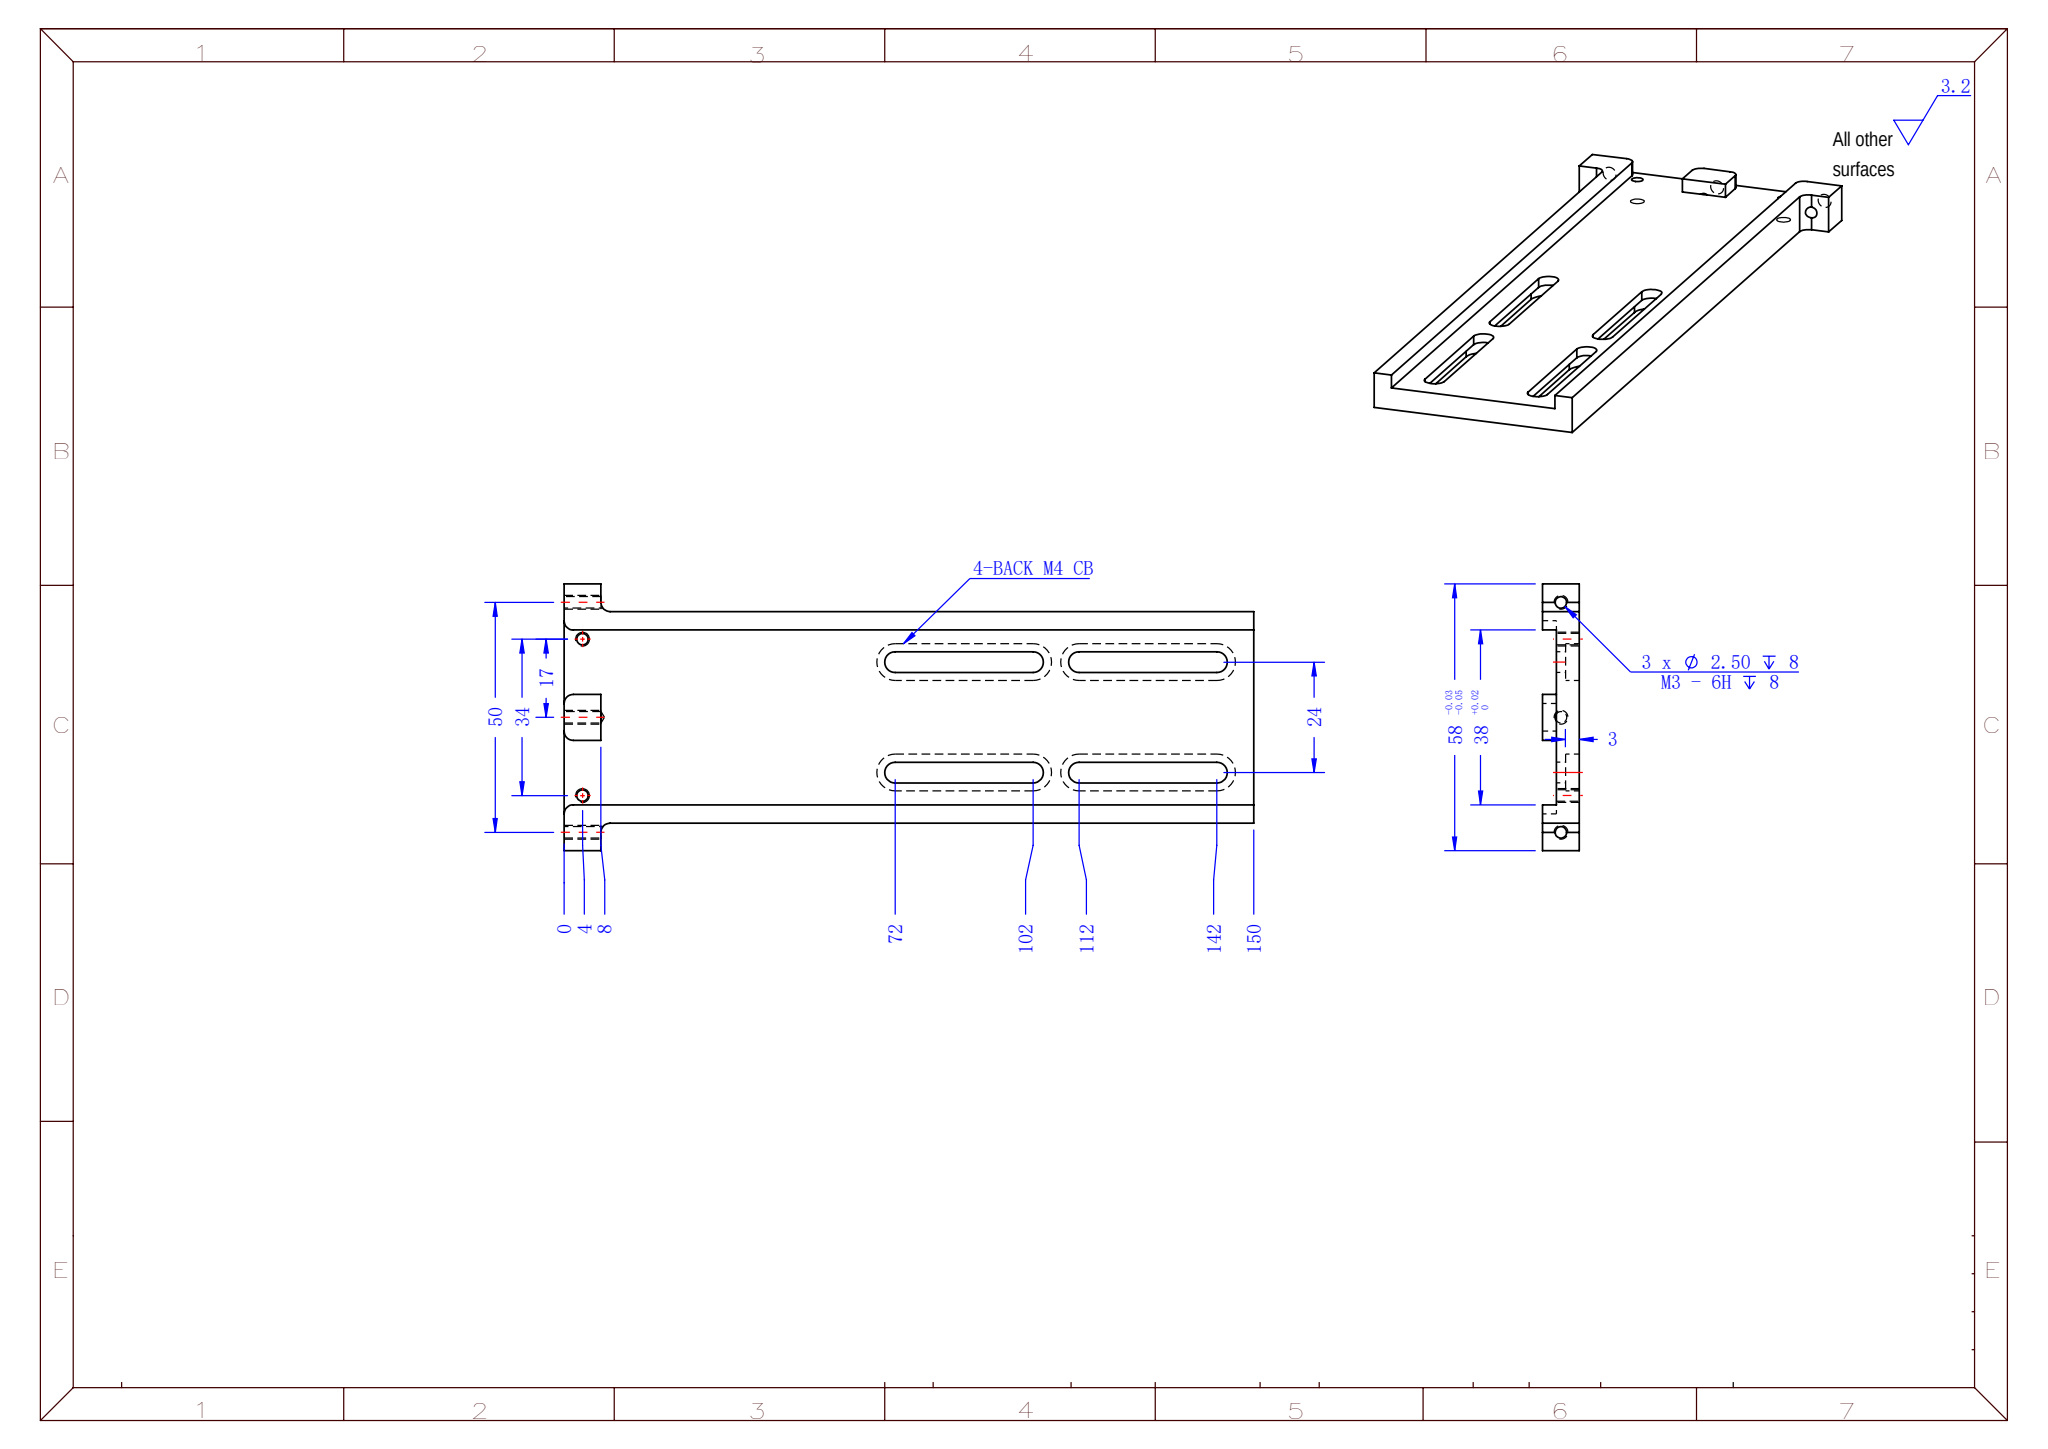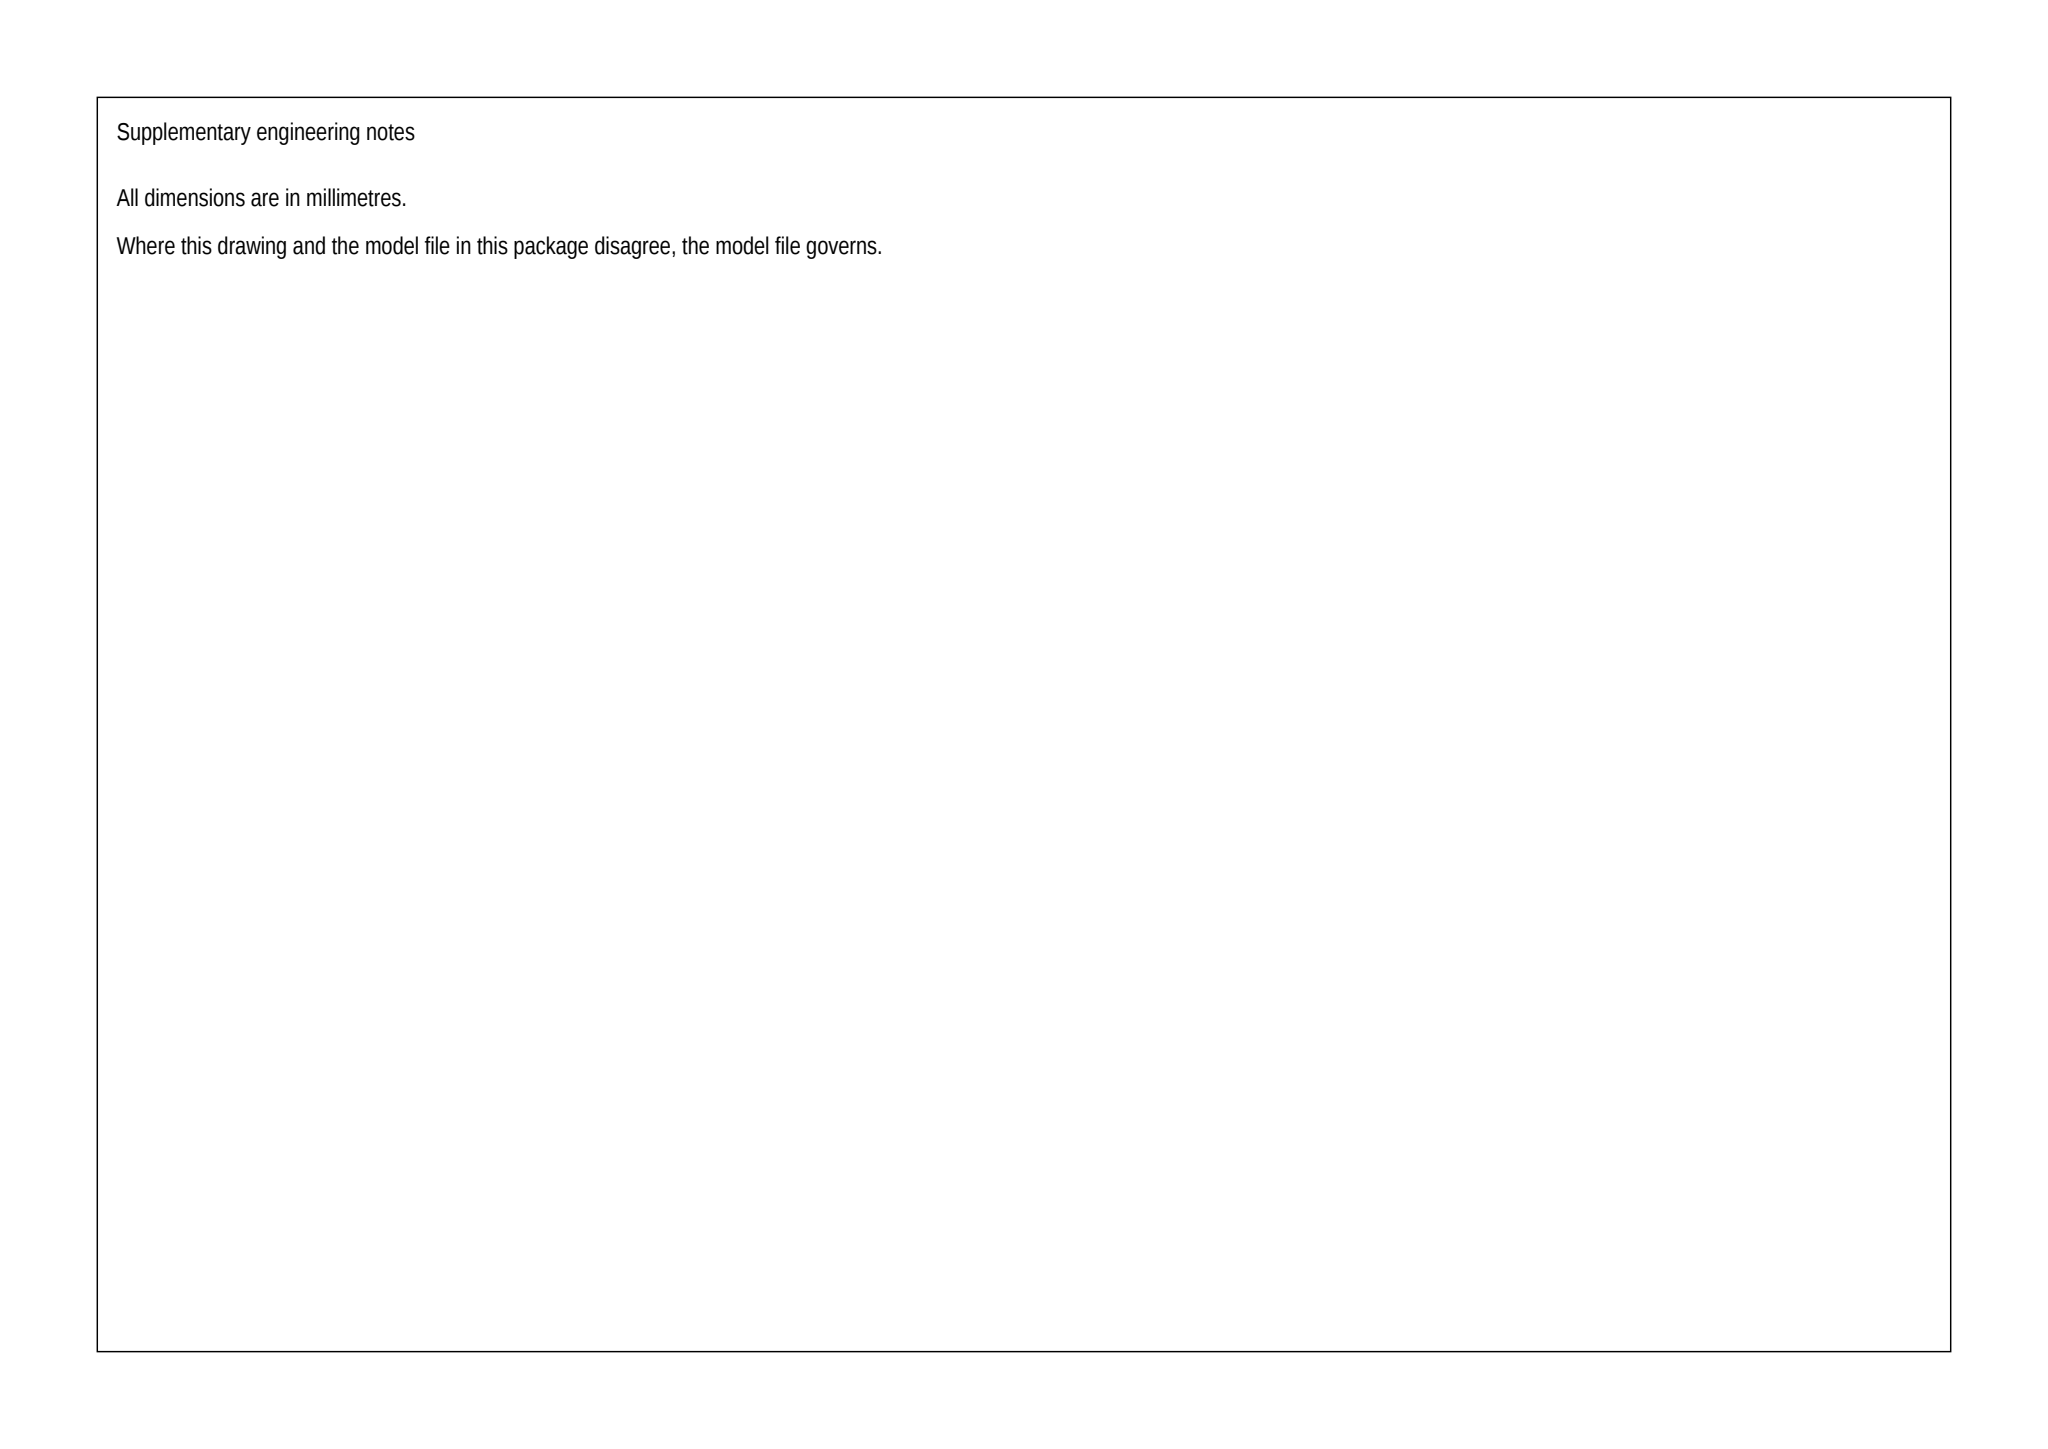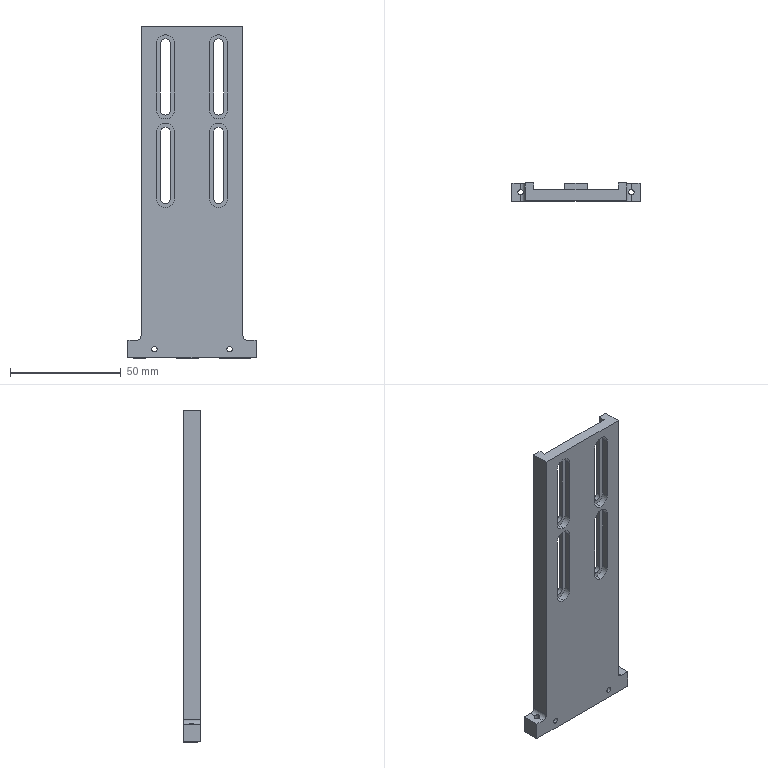Part | SolidWorks | mm | 1 solid | 80 faces | box 58 x 8 x 150 mm | volume 34252 mm3 | cylinder 40 | plane 38 | cone 2 | commonest cylinder face diameters 8 x12 4.5 x12 2.5 x10 4 x6
Drawing notes:
2X R2 FILLET AT EAR/BODY STEP, 10 FROM 0 DATUM, THRU 8 THK | from the solid: concave arcs dia 4.0 (R2), axis y, at (x=4,z=10) and (x=54,z=10), from y0 to y8, 90 deg - inside fillets where 58 wide ears step down to 46 wide body